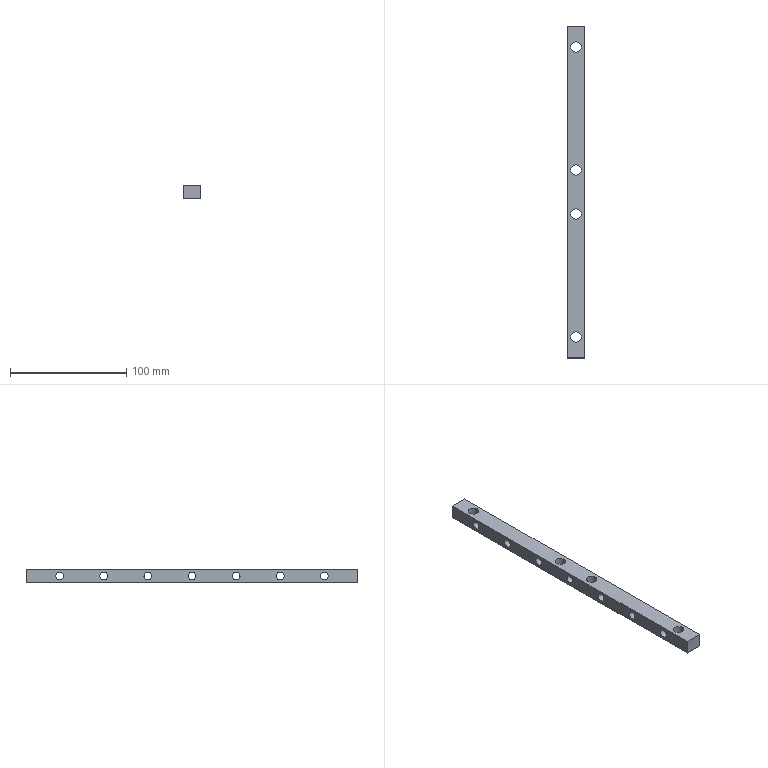Component | NX | FIXED_PLATE_9 | 1 solid | 17 faces | volume 44613 mm3 | cylinder 11 | plane 6 | commonest cylinder face diameters 6.8 x7 9 x4